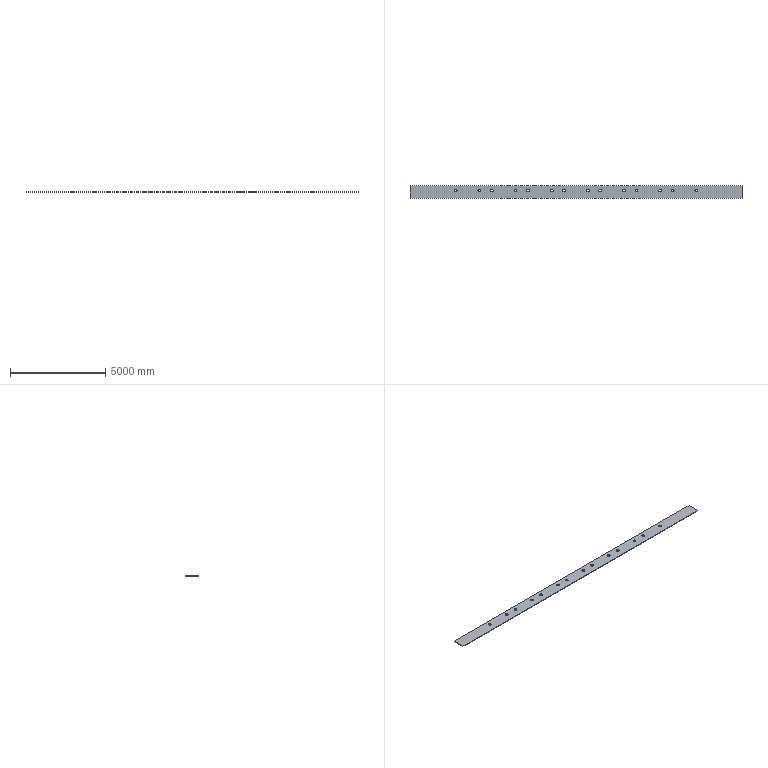Component | SolidWorks | ElectromagneticBeamTopPlate-1 | 1 solid | 34 faces | volume 332657987 mm3 | cylinder 28 | plane 6 | commonest cylinder face diameters 150 x28 | material Plain Carbon Steel